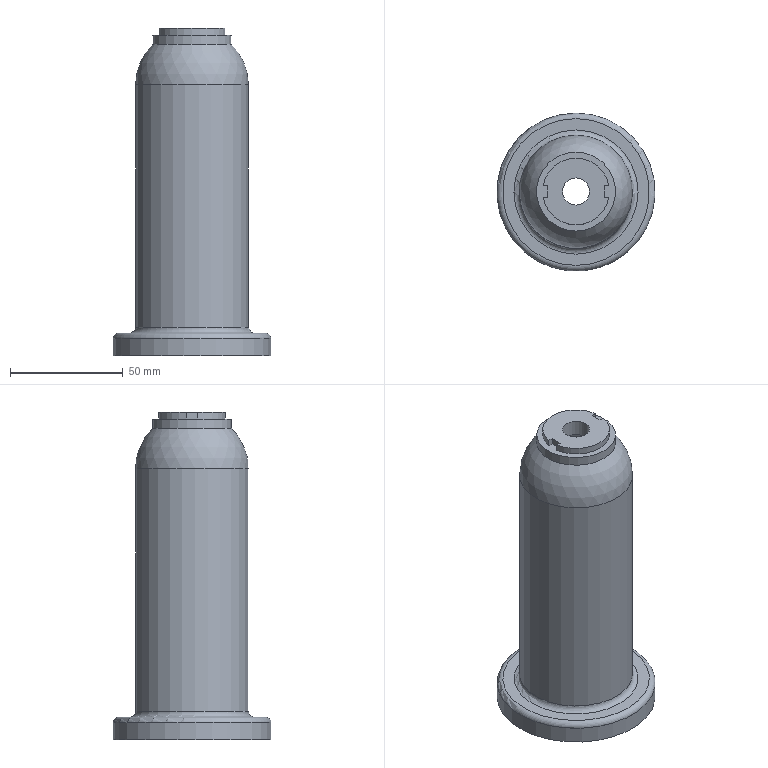Component | NX | VALVE_BONNET | 1 solid | 25 faces | volume 116508 mm3 | plane 12 | cylinder 8 | torus 3 | sphere 2 | commonest cylinder face diameters 29.58 x2 70 x1 50 x1 35 x1 40 x1 60 x1 12 x1